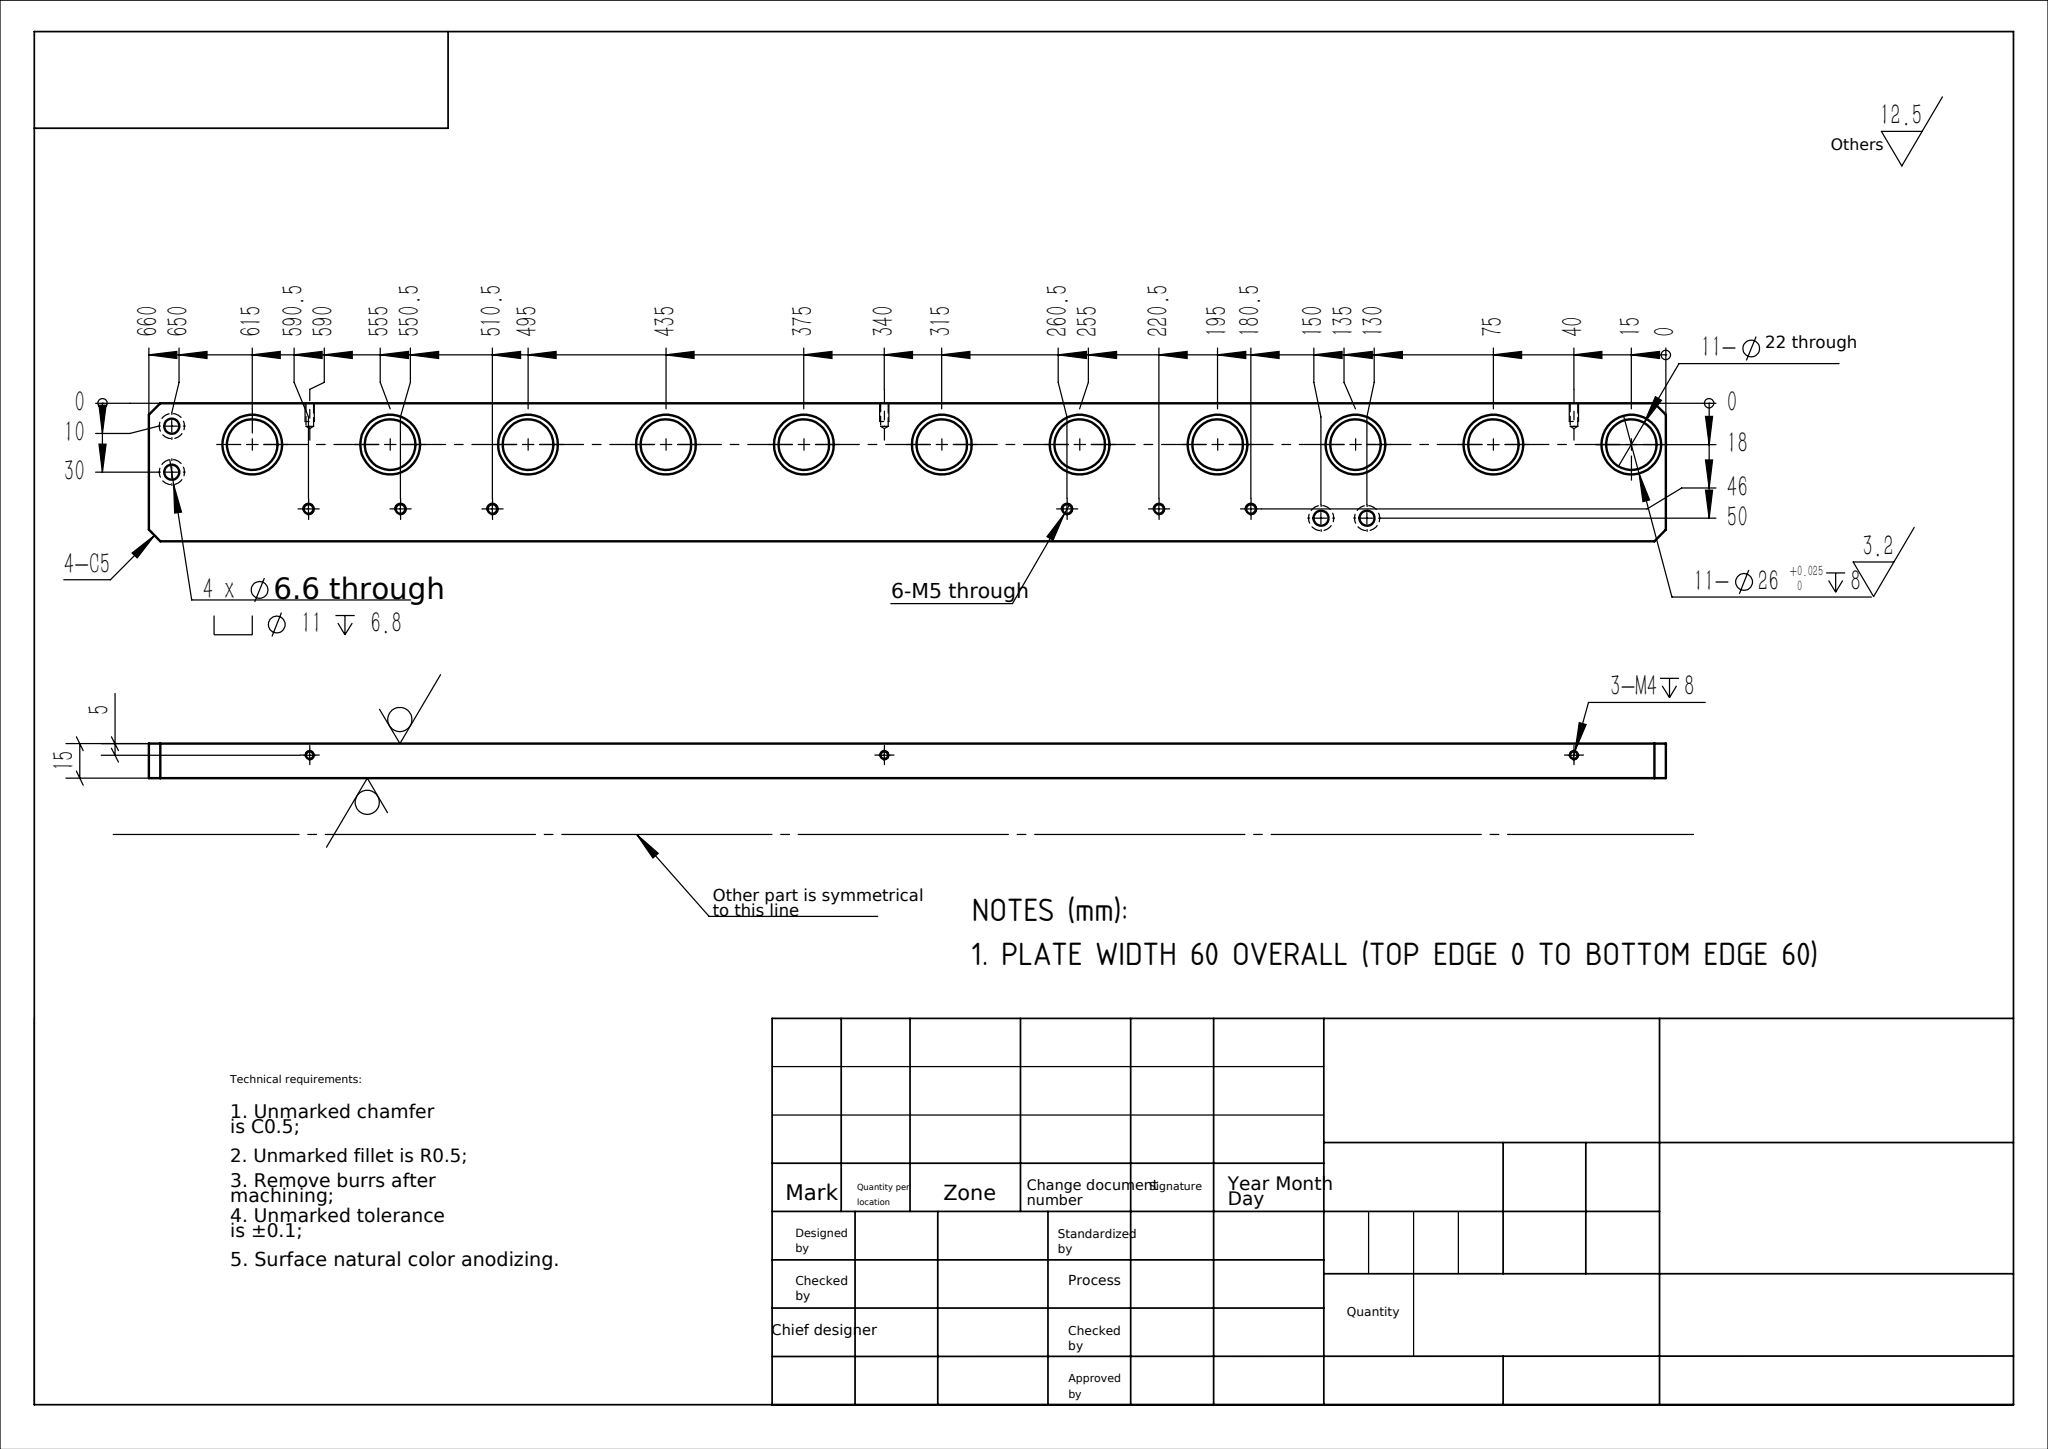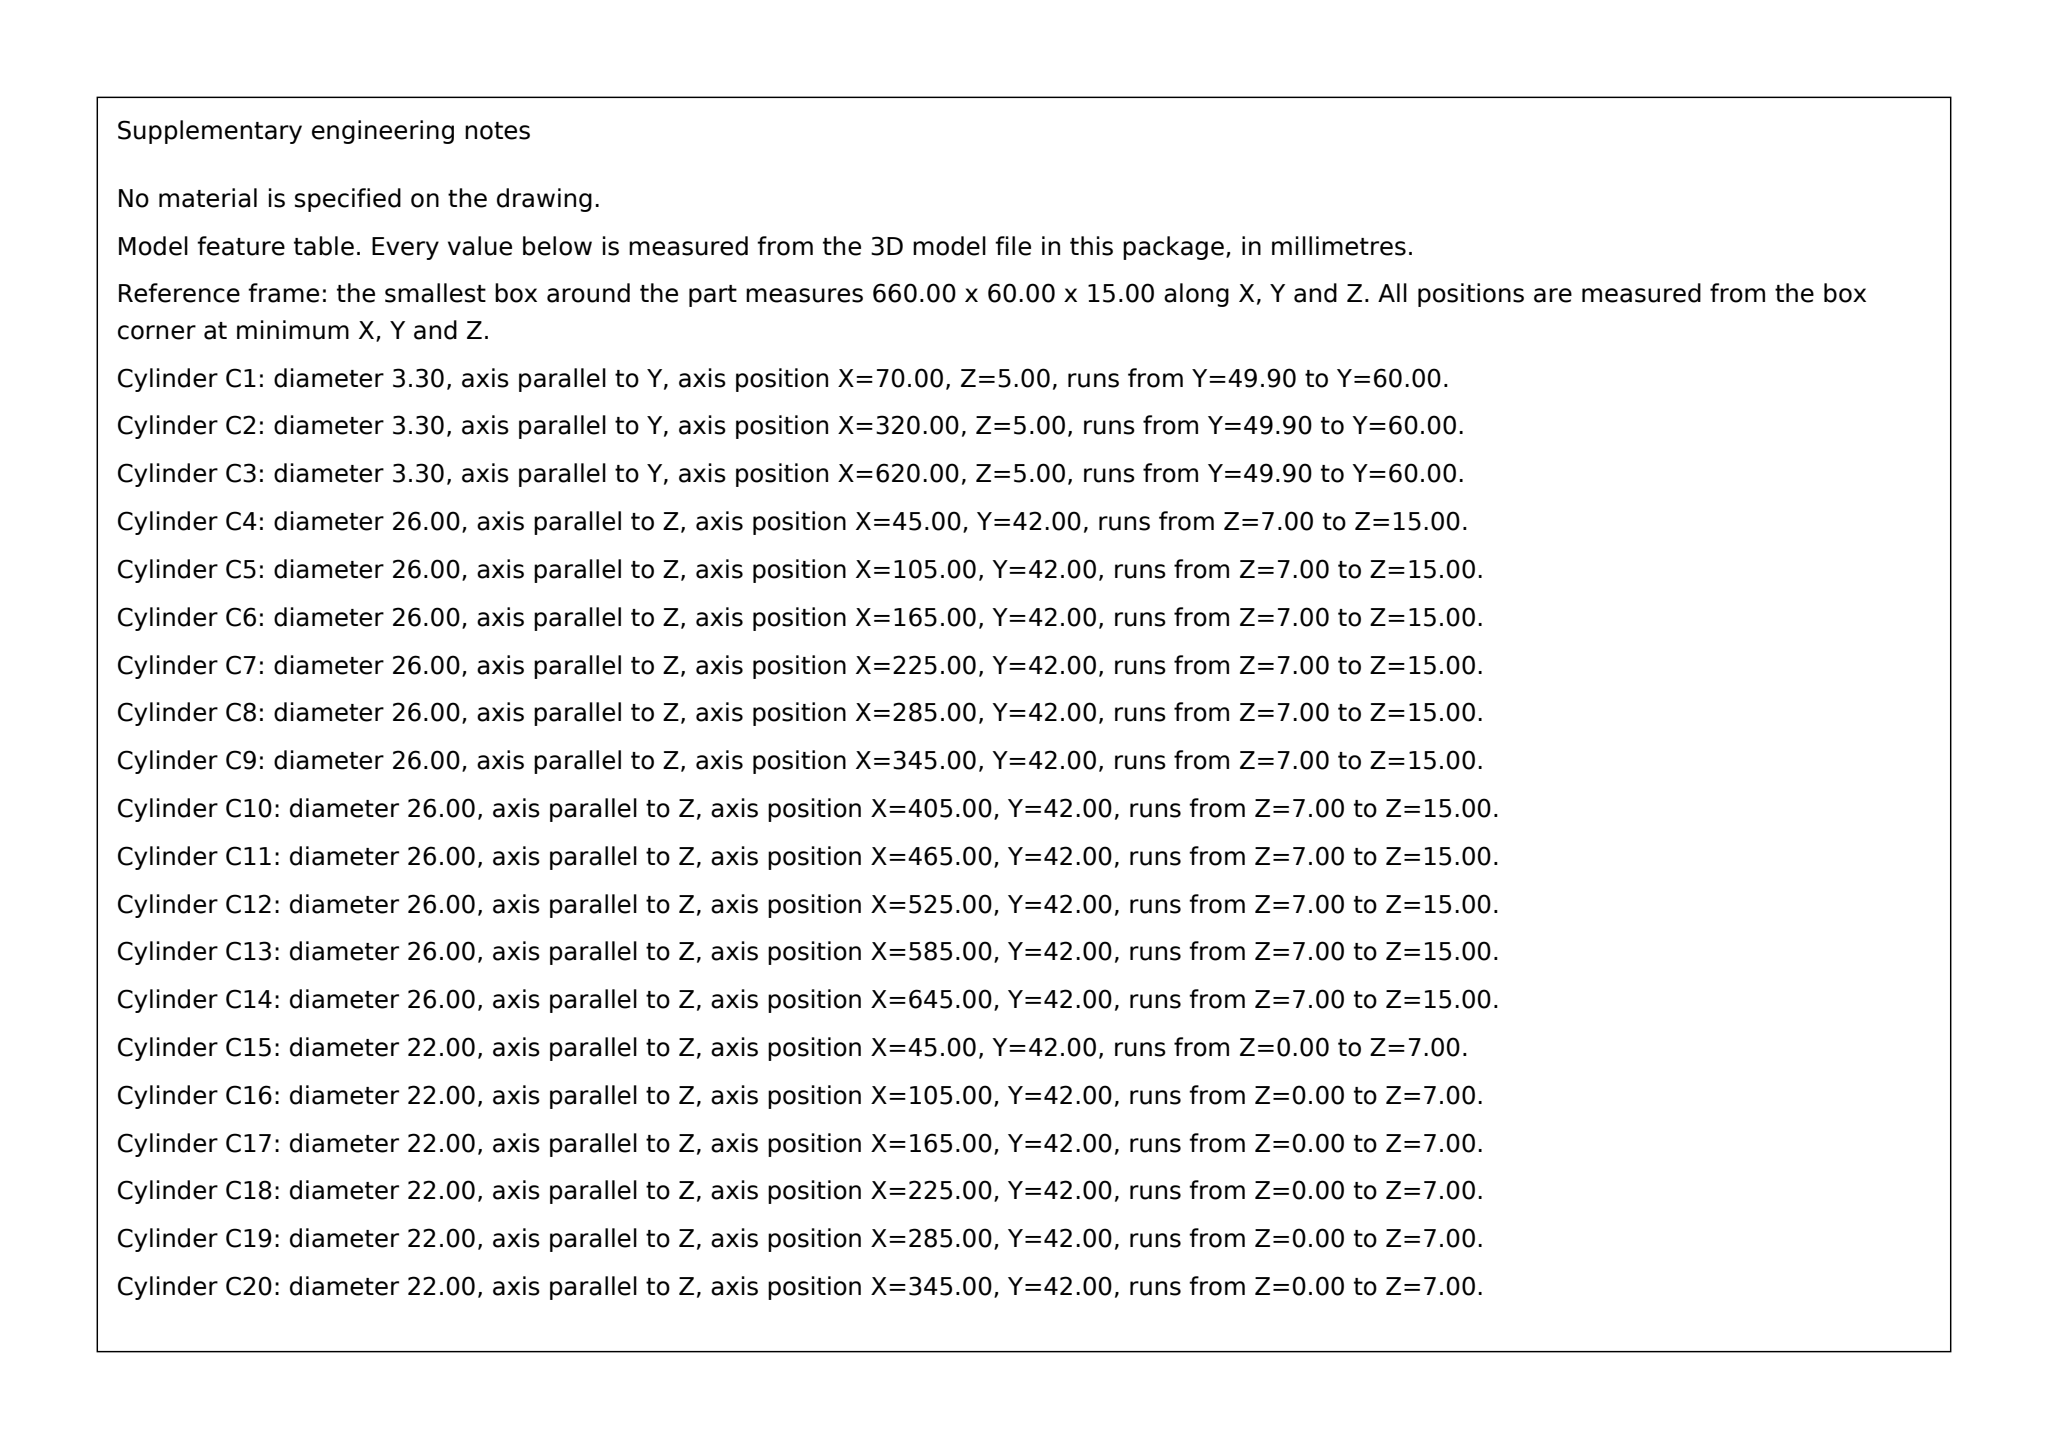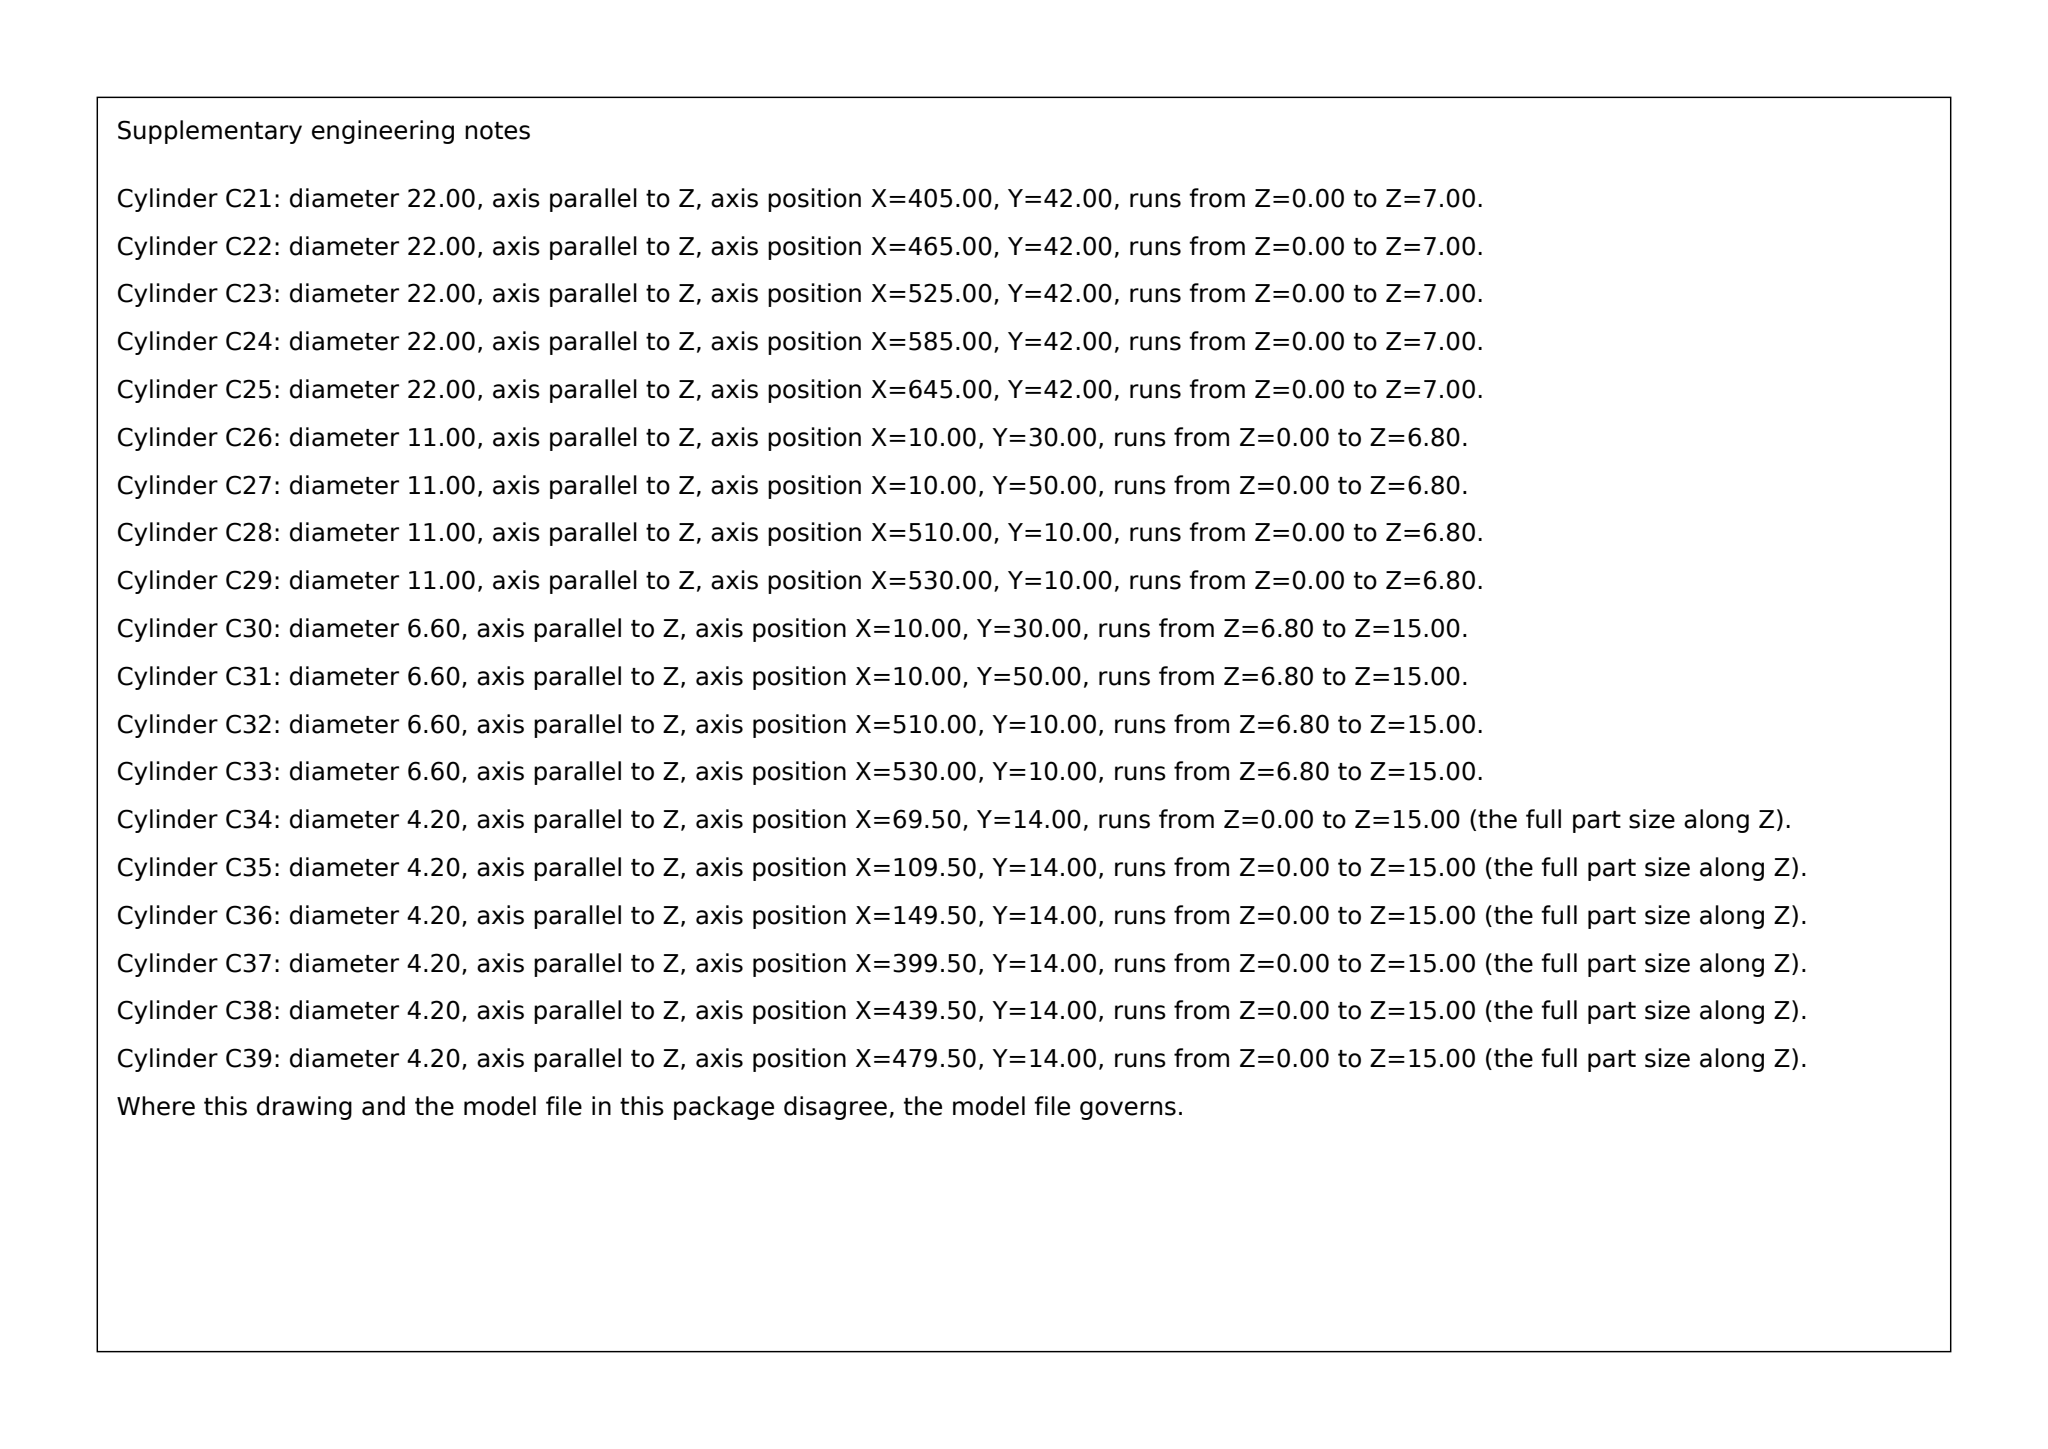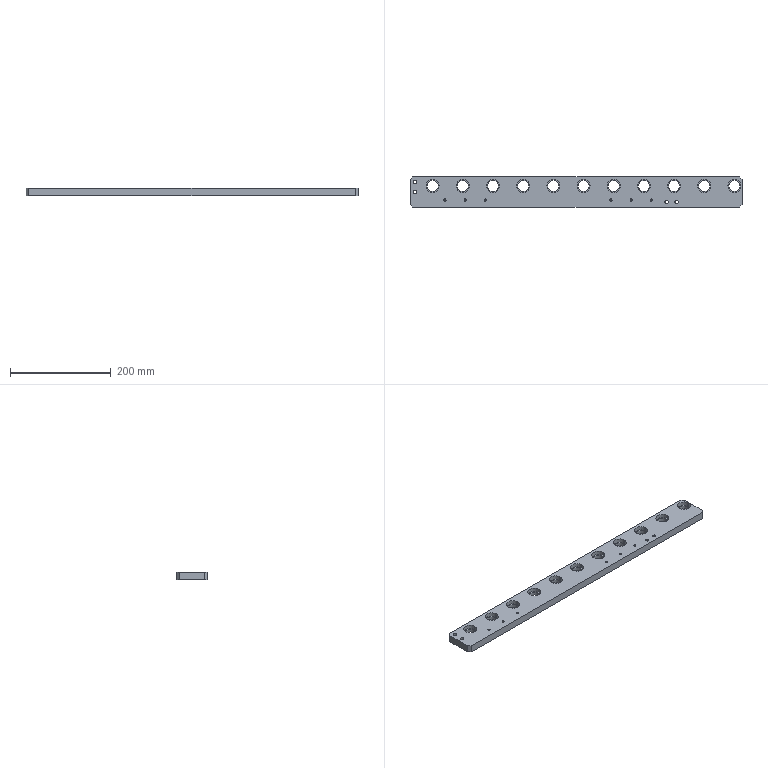Part | SolidWorks | mm | 1 solid | 109 faces | box 660 x 60 x 15 mm | volume 512036 mm3 | cylinder 78 | plane 25 | cone 6 | commonest cylinder face diameters 22 x22 26 x22 4.2 x12 11 x8 6.6 x8 3.3 x6
Drawing notes:
PLATE WIDTH 60 OVERALL (TOP EDGE 0 TO BOTTOM EDGE 60) | from the solid: bbox_xyz y=60.0; axis_planes y=0.0 and y=60.0
build123d program:
from build123d import *

# Parameters (mm, degrees)
SKETCH1_W                                            = 660
SKETCH1_H                                            = 60
BOSS_EXTRUDE1_DEPTH                                  = 15
SKETCH2_R                                            = 13
CUT_EXTRUDE1_DEPTH                                   = 8
SKETCH3_R                                            = 11
CUT_EXTRUDE2_DEPTH                                   = 332.7
LPATTERN1_COUNT                                      = 11
LPATTERN1_PITCH                                      = 60
CHAMFER1_SIZE                                        = 5
M4_TAPPED_HOLE1_D                                    = 3.3
M4_TAPPED_HOLE1_DEPTH                                = 10.1
M4_TAPPED_HOLE1_TIP                                  = 0.9914
HOLE_SIZE_ACCORDING_TO_HEXAGON_SOCKET_HE_D           = 6.6
HOLE_SIZE_ACCORDING_TO_HEXAGON_SOCKET_HE_CBORE_D     = 11
HOLE_SIZE_ACCORDING_TO_HEXAGON_SOCKET_HE_CBORE_DEPTH = 6.8
M5_TAPPED_HOLE1_D                                    = 4.2


with BuildPart() as part:
    # Sketch1 → Boss-Extrude1 (new body)
    with BuildSketch(Plane.XY):
        Rectangle(SKETCH1_W, SKETCH1_H)
    extrude(amount=BOSS_EXTRUDE1_DEPTH)

    # Sketch2 → Cut-Extrude1 (cut)
    with BuildSketch(Plane.XY.offset(15)):
        with Locations((315, 12)):
            Circle(SKETCH2_R)
    cut_extrude1 = extrude(amount=-CUT_EXTRUDE1_DEPTH, mode=Mode.SUBTRACT)

    # Sketch3 → Cut-Extrude2 (cut, through all)
    with BuildSketch(Plane.XY.offset(15)):
        with Locations((315, 12)):
            Circle(SKETCH3_R)
    cut_extrude2 = extrude(amount=-CUT_EXTRUDE2_DEPTH, mode=Mode.SUBTRACT)

    # LPattern1: Cut-Extrude1, Cut-Extrude2 ×11
    with Locations(*[(-i * LPATTERN1_PITCH, 0, 0) for i in range(1, LPATTERN1_COUNT)]):
        add(cut_extrude1, mode=Mode.SUBTRACT)
        add(cut_extrude2, mode=Mode.SUBTRACT)

    # Chamfer1
    chamfer1_edges = [part.edges().sort_by_distance(p)[0] for p in [
        (330, -30, 7.5),
        (-330, -30, 7.5),
        (-330, 30, 7.5),
        (330, 30, 7.5),
    ]]
    chamfer(chamfer1_edges, length=CHAMFER1_SIZE)

    # M4 Tapped Hole1
    with Locations(Plane(origin=(0, 30, 0), x_dir=(1, 0, 0), z_dir=(0, 1, 0))):
        with Locations((290, -5), (-10, -5), (-260, -5)):
            Hole(M4_TAPPED_HOLE1_D / 2, depth=M4_TAPPED_HOLE1_DEPTH)
            with Locations((0, 0, -(M4_TAPPED_HOLE1_DEPTH + M4_TAPPED_HOLE1_TIP / 2))):  # 118° drill point
                Cone(0, M4_TAPPED_HOLE1_D / 2, M4_TAPPED_HOLE1_TIP, mode=Mode.SUBTRACT)

    # Hole Size_According to_Hexagon Socket He (through all)
    with Locations(Plane(origin=(0, 0, 0), x_dir=(-1, 0, 0), z_dir=(0, 0, -1))):
        with Locations((320, 20), (320, 0), (-200, -20), (-180, -20)):
            CounterBoreHole(HOLE_SIZE_ACCORDING_TO_HEXAGON_SOCKET_HE_D / 2, HOLE_SIZE_ACCORDING_TO_HEXAGON_SOCKET_HE_CBORE_D / 2, HOLE_SIZE_ACCORDING_TO_HEXAGON_SOCKET_HE_CBORE_DEPTH)

    # M5 Tapped Hole1 (through all)
    with Locations(Plane(origin=(0, 0, 0), x_dir=(-1, 0, 0), z_dir=(0, 0, -1))):
        with Locations((260.5, -16), (220.5, -16), (180.5, -16), (-69.5, -16), (-109.5, -16), (-149.5, -16)):
            Hole(M5_TAPPED_HOLE1_D / 2)


solid = part.part